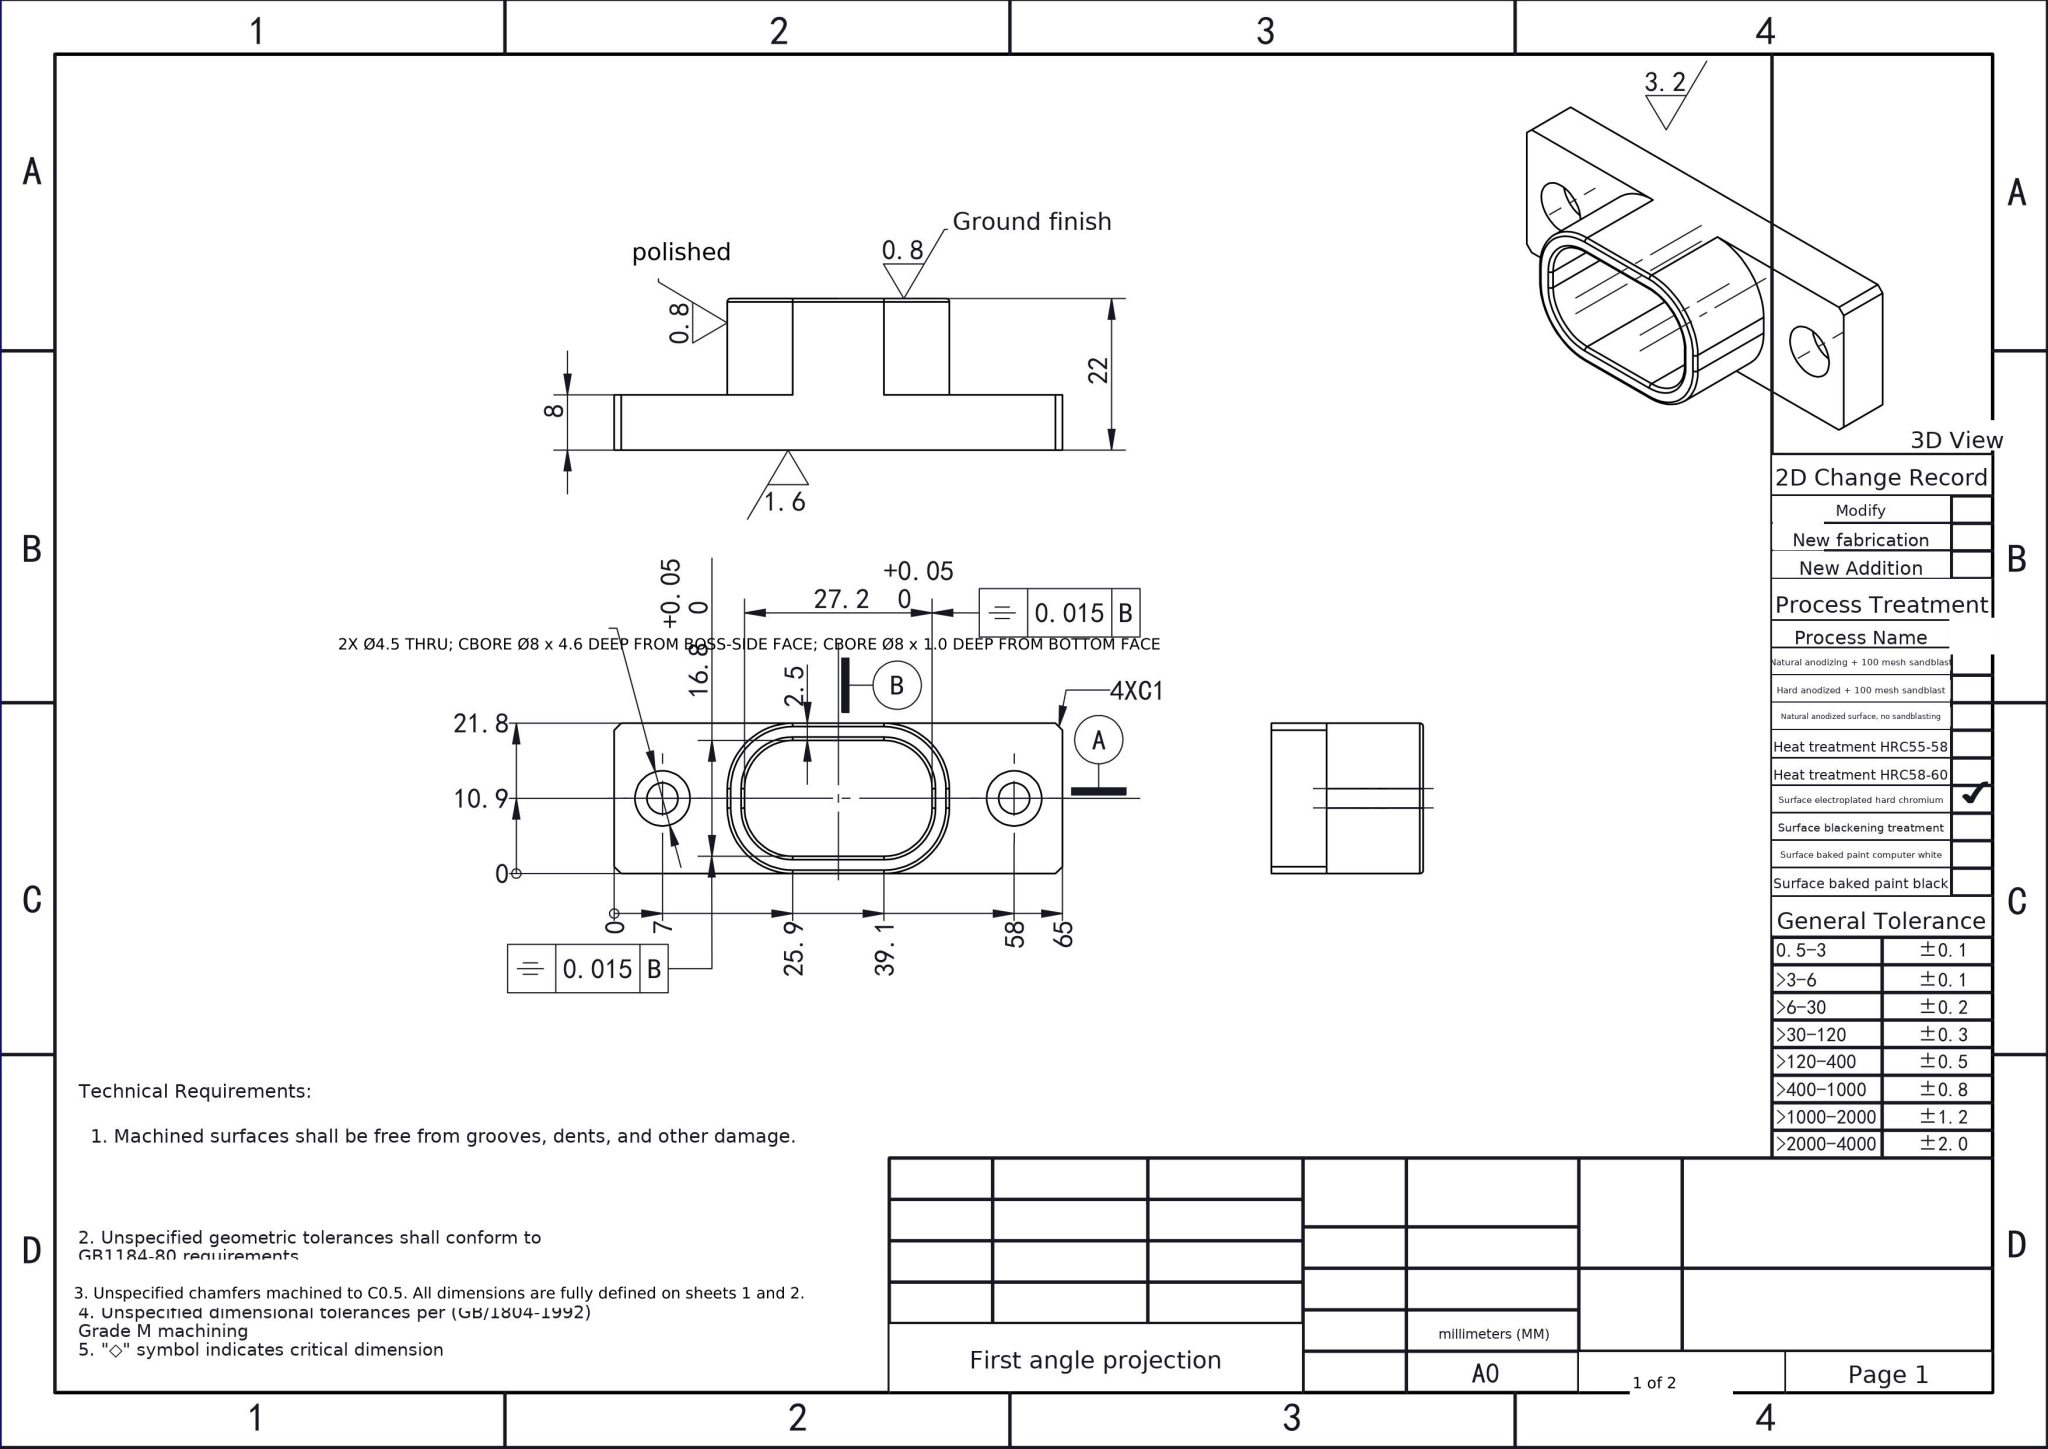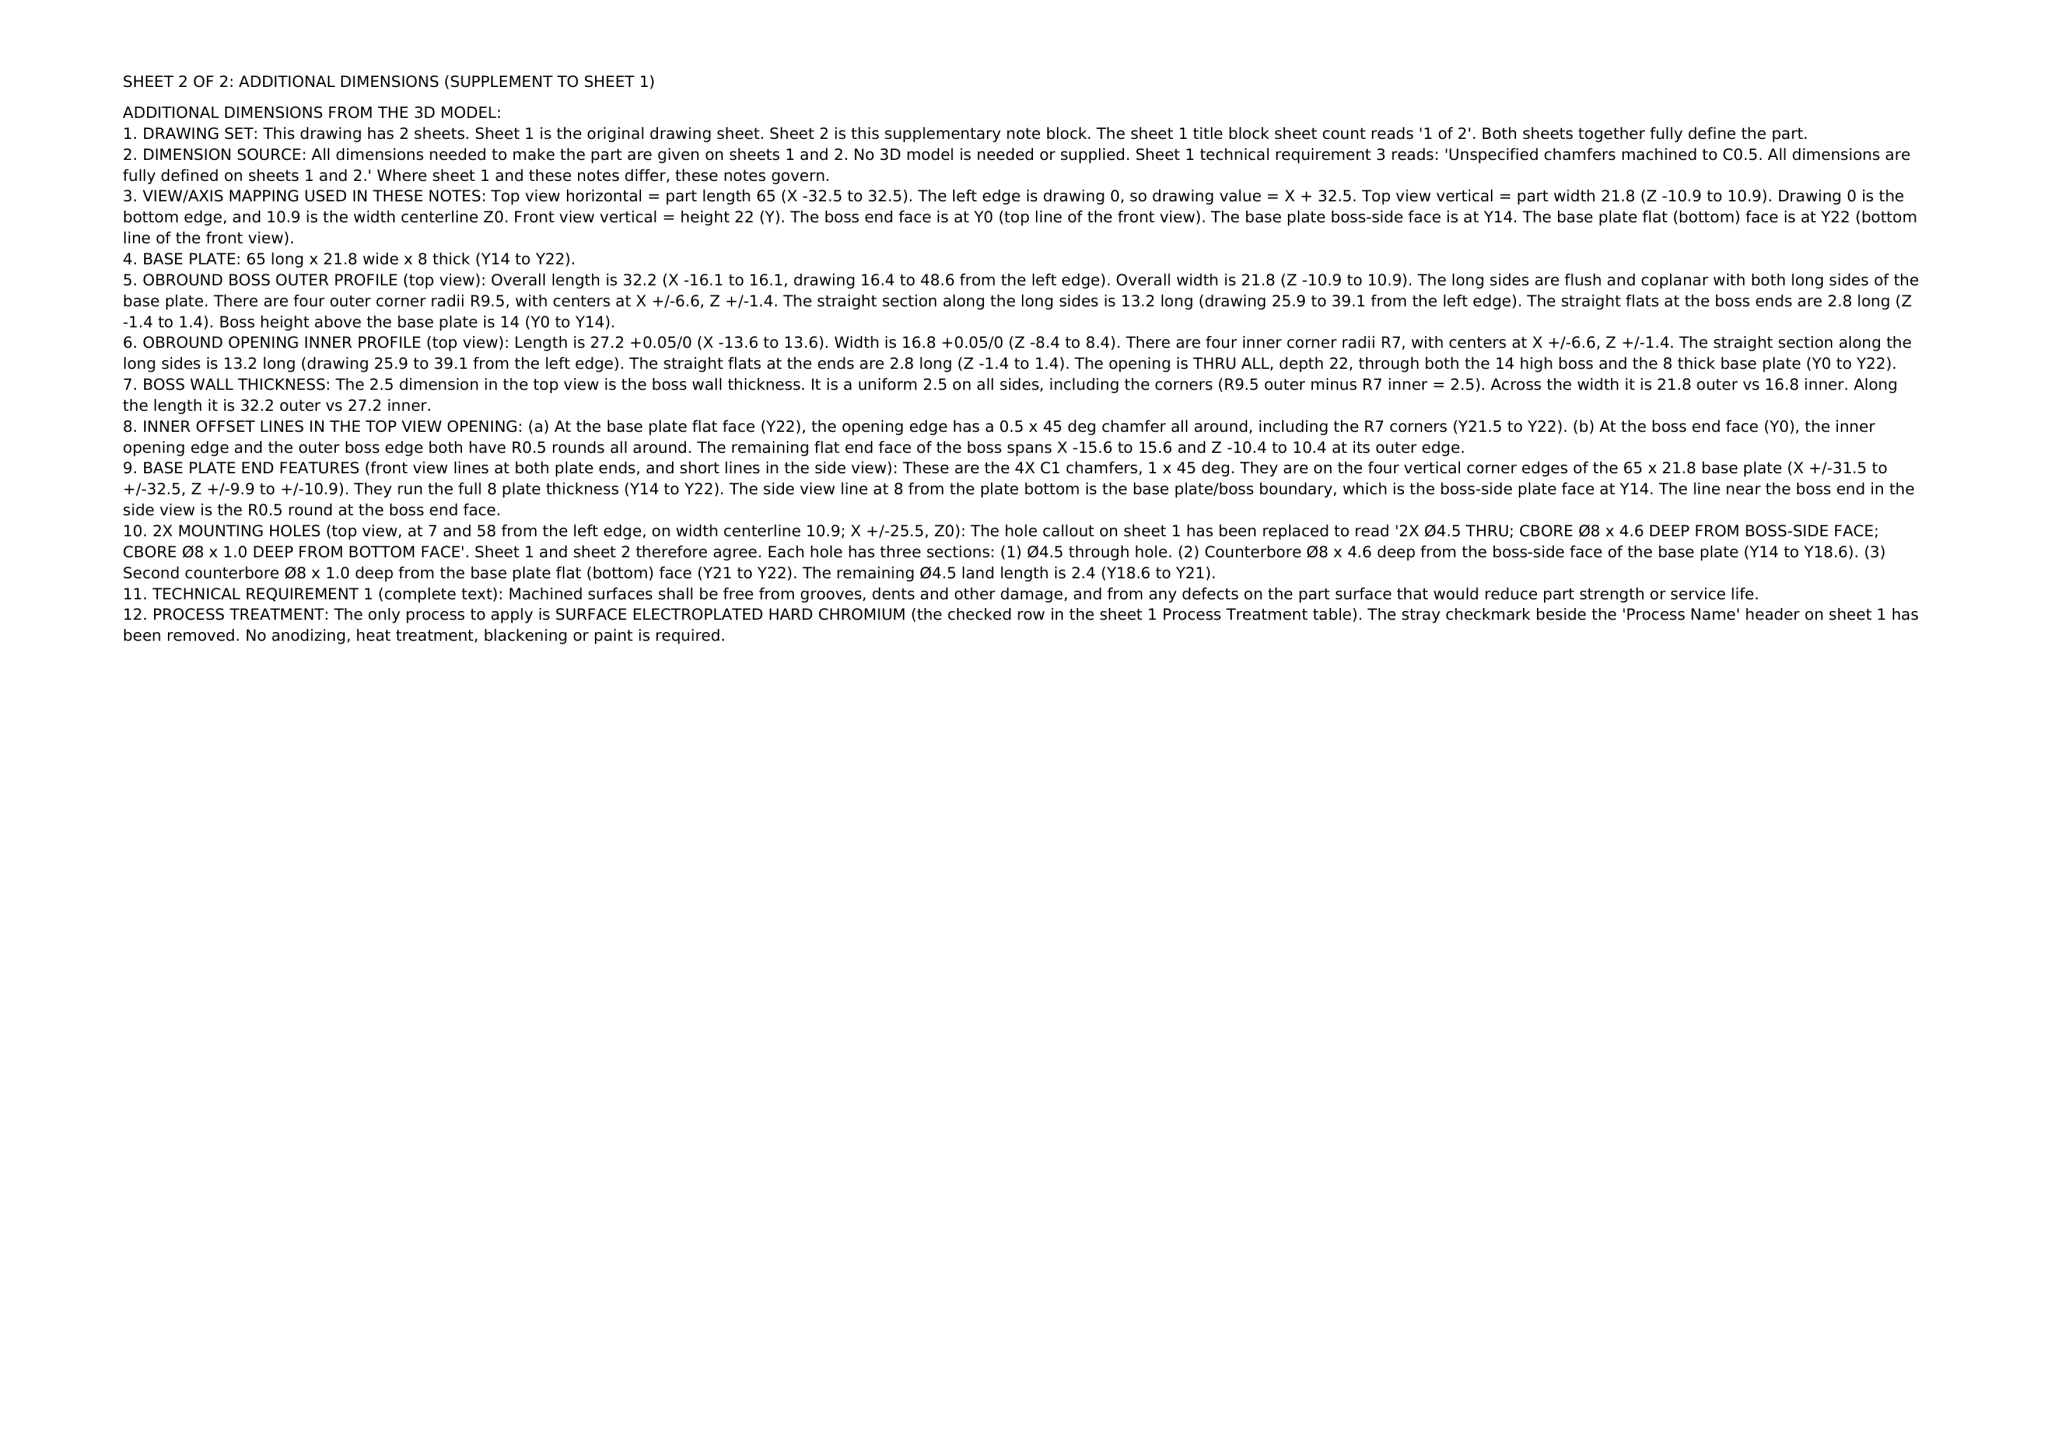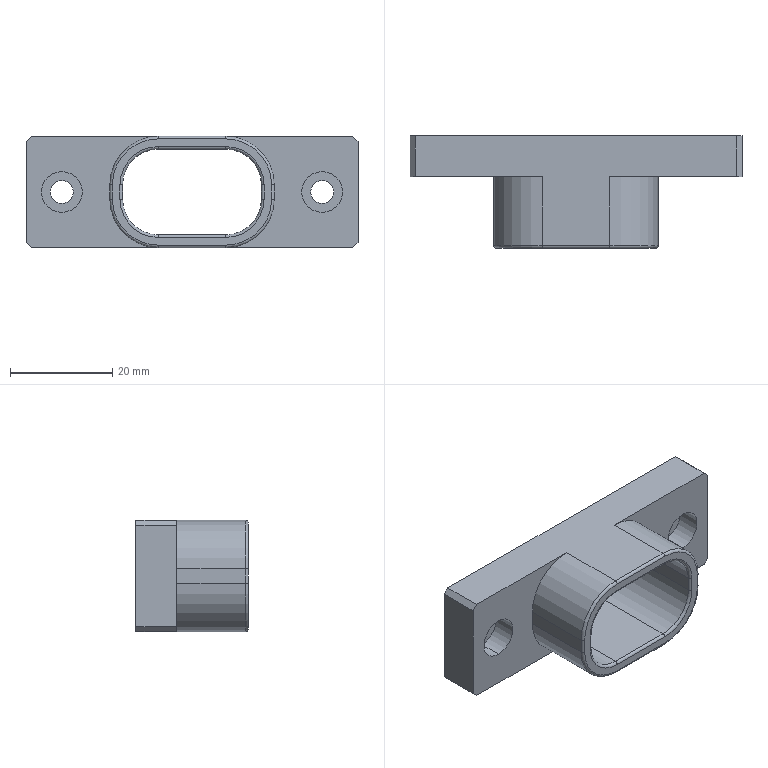Part | NX | mm | Oval-Bore Flanged Mount | 1 solid | 66 faces | box 65 x 22 x 21.8 mm | volume 10277 mm3 | cylinder 28 | plane 26 | torus 8 | cone 4 | commonest cylinder face diameters 8 x8 1 x8 4.5 x4 19 x4 14 x4